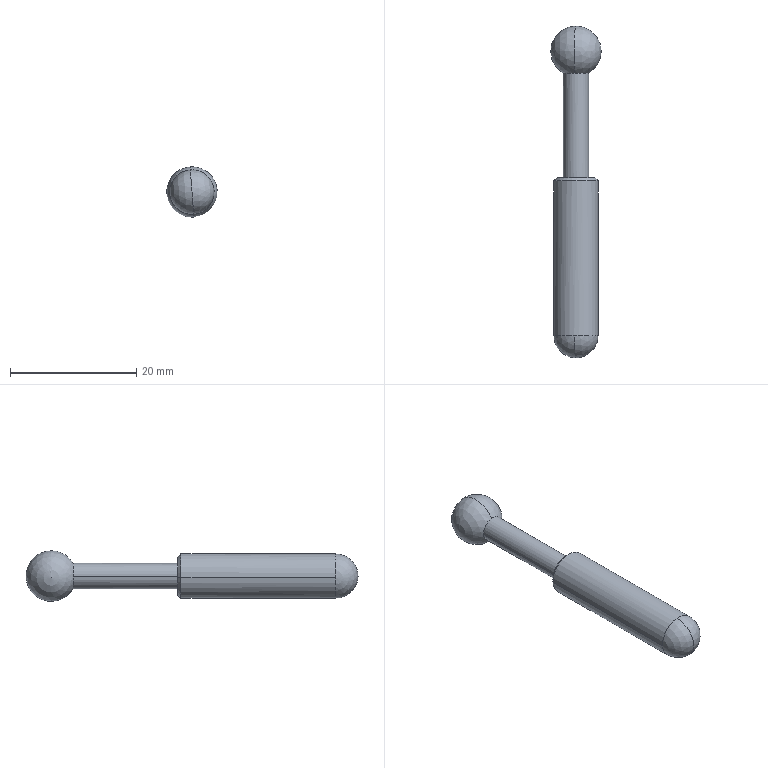Component | SolidWorks | GuidePost-1 | 1 solid | 11 faces | box 8 x 52.5 x 8 mm | volume 1522 mm3 | cylinder 4 | sphere 4 | cone 2 | plane 1 | commonest cylinder face diameters 4 x2 7 x2
build123d program:
from build123d import *

# Parameters (mm, degrees)
CHAMFER1_SIZE = 0.5


with BuildPart() as part:
    # Sketch1 → Revolve1 (revolve)
    with BuildSketch(Plane(origin=(0, 0, 0), x_dir=(0, 0, -1), z_dir=(1, 0, 0))):
        with BuildLine():
            Line((3.464, 2), (20, 2))
            Line((20, 2), (20, 3.5))
            Line((20, 3.5), (45, 3.5))
            ThreePointArc((45, 3.5), (47.475, 2.475), (48.5, 0))
            Line((48.5, 0), (-4, 0))
            ThreePointArc((-4, 0), (-1.035, 3.864), (3.464, 2))
        make_face()
    revolve(axis=Axis((0, 0, 4), (0, 0, -1)))

    # Chamfer1
    chamfer1_edges = [part.edges().sort_by_distance(p)[0] for p in [
        (0, -3.5, -20),
    ]]
    chamfer(chamfer1_edges, length=CHAMFER1_SIZE)


solid = part.part

# Placed as in the assembly
solid = solid.moved(Location((111.546, 64.028, 491.671), (-90, 0, 0)))
STEP:
#1=COLOUR_RGB('',0.7922,0.8196,0.9333);
#2=FILL_AREA_STYLE_COLOUR('',#1);
#3=FILL_AREA_STYLE('',(#2));
#4=SURFACE_STYLE_FILL_AREA(#3);
#5=SURFACE_SIDE_STYLE('',(#4));
#6=SURFACE_STYLE_USAGE(.BOTH.,#5);
#7=PRESENTATION_STYLE_ASSIGNMENT((#6));
#8=CARTESIAN_POINT('',(4.274,1.733,19.348));
#9=VERTEX_POINT('',#8);
#10=CARTESIAN_POINT('',(4.509,1.733,19.366));
#11=VERTEX_POINT('',#10);
#12=CARTESIAN_POINT('',(4.392,1.733,19.357));
#13=DIRECTION('',(0.,1.,0.));
#14=DIRECTION('',(0.9973,0.,0.07369));
#15=AXIS2_PLACEMENT_3D('',#12,#13,#14);
#16=CIRCLE('',#15,0.1181);
#17=EDGE_CURVE('',#9,#11,#16,.T.);
#18=ORIENTED_EDGE('',*,*,#17,.F.);
#19=CARTESIAN_POINT('',(4.254,1.714,19.347));
#20=VERTEX_POINT('',#19);
#21=CARTESIAN_POINT('',(4.274,1.733,19.348));
#22=DIRECTION('',(-0.7052,-0.7071,-0.05211));
#23=VECTOR('',#22,39.37);
#24=LINE('',#21,#23);
#25=EDGE_CURVE('',#9,#20,#24,.T.);
#26=ORIENTED_EDGE('',*,*,#25,.T.);
#27=CARTESIAN_POINT('',(4.529,1.714,19.367));
#28=VERTEX_POINT('',#27);
#29=CARTESIAN_POINT('',(4.392,1.714,19.357));
#30=DIRECTION('',(-0.,-1.,-0.));
#31=DIRECTION('',(0.9973,0.,0.07369));
#32=AXIS2_PLACEMENT_3D('',#29,#30,#31);
#33=CIRCLE('',#32,0.1378);
#34=EDGE_CURVE('',#28,#20,#33,.T.);
#35=ORIENTED_EDGE('',*,*,#34,.F.);
#36=CARTESIAN_POINT('',(4.509,1.733,19.366));
#37=DIRECTION('',(0.7052,-0.7071,0.05211));
#38=VECTOR('',#37,39.37);
#39=LINE('',#36,#38);
#40=EDGE_CURVE('',#11,#28,#39,.T.);
#41=ORIENTED_EDGE('',*,*,#40,.F.);
#42=EDGE_LOOP('',(#18,#26,#35,#41));
#43=FACE_OUTER_BOUND('',#42,.T.);
#44=CARTESIAN_POINT('',(4.392,1.733,19.357));
#45=DIRECTION('',(-0.,-1.,-0.));
#46=DIRECTION('',(0.9973,0.,0.07369));
#47=AXIS2_PLACEMENT_3D('',#44,#45,#46);
#48=CONICAL_SURFACE('',#47,0.1181,0.7854);
#49=ADVANCED_FACE('',(#43),#48,.T.);
#50=CARTESIAN_POINT('',(4.313,1.733,19.351));
#51=VERTEX_POINT('',#50);
#52=CARTESIAN_POINT('',(4.47,1.733,19.363));
#53=VERTEX_POINT('',#52);
#54=CARTESIAN_POINT('',(4.392,1.733,19.357));
#55=DIRECTION('',(0.,1.,0.));
#56=DIRECTION('',(-0.9973,0.,-0.07369));
#57=AXIS2_PLACEMENT_3D('',#54,#55,#56);
#58=CIRCLE('',#57,0.07874);
#59=EDGE_CURVE('',#51,#53,#58,.T.);
#60=ORIENTED_EDGE('',*,*,#59,.T.);
#61=CARTESIAN_POINT('',(4.47,2.384,19.363));
#62=VERTEX_POINT('',#61);
#63=CARTESIAN_POINT('',(4.47,2.678,19.363));
#64=DIRECTION('',(0.,1.,0.));
#65=VECTOR('',#64,39.37);
#66=LINE('',#63,#65);
#67=EDGE_CURVE('',#53,#62,#66,.T.);
#68=ORIENTED_EDGE('',*,*,#67,.T.);
#69=CARTESIAN_POINT('',(4.386,2.384,19.436));
#70=VERTEX_POINT('',#69);
#71=CARTESIAN_POINT('',(4.392,2.384,19.357));
#72=DIRECTION('',(0.,1.,0.));
#73=DIRECTION('',(-0.9973,0.,-0.07369));
#74=AXIS2_PLACEMENT_3D('',#71,#72,#73);
#75=CIRCLE('',#74,0.07874);
#76=EDGE_CURVE('',#70,#62,#75,.T.);
#77=ORIENTED_EDGE('',*,*,#76,.F.);
#78=CARTESIAN_POINT('',(4.313,2.384,19.351));
#79=VERTEX_POINT('',#78);
#80=CARTESIAN_POINT('',(4.392,2.384,19.357));
#81=DIRECTION('',(0.,1.,0.));
#82=DIRECTION('',(-0.9973,0.,-0.07369));
#83=AXIS2_PLACEMENT_3D('',#80,#81,#82);
#84=CIRCLE('',#83,0.07874);
#85=EDGE_CURVE('',#79,#70,#84,.T.);
#86=ORIENTED_EDGE('',*,*,#85,.F.);
#87=CARTESIAN_POINT('',(4.313,2.678,19.351));
#88=DIRECTION('',(0.,1.,0.));
#89=VECTOR('',#88,39.37);
#90=LINE('',#87,#89);
#91=EDGE_CURVE('',#51,#79,#90,.T.);
#92=ORIENTED_EDGE('',*,*,#91,.F.);
#93=EDGE_LOOP('',(#60,#68,#77,#86,#92));
#94=FACE_OUTER_BOUND('',#93,.T.);
#95=CARTESIAN_POINT('',(4.392,2.678,19.357));
#96=DIRECTION('',(0.,1.,0.));
#97=DIRECTION('',(-0.9973,0.,-0.07369));
#98=AXIS2_PLACEMENT_3D('',#95,#96,#97);
#99=CYLINDRICAL_SURFACE('',#98,0.07874);
#100=ADVANCED_FACE('',(#94),#99,.T.);
#101=CARTESIAN_POINT('',(4.381,0.7492,19.495));
#102=VERTEX_POINT('',#101);
#103=CARTESIAN_POINT('',(4.529,0.7492,19.367));
#104=VERTEX_POINT('',#103);
#105=CARTESIAN_POINT('',(4.392,0.7492,19.357));
#106=DIRECTION('',(0.,1.,0.));
#107=DIRECTION('',(-0.9973,0.,-0.07369));
#108=AXIS2_PLACEMENT_3D('',#105,#106,#107);
#109=CIRCLE('',#108,0.1378);
#110=EDGE_CURVE('',#102,#104,#109,.T.);
#111=ORIENTED_EDGE('',*,*,#110,.T.);
#112=CARTESIAN_POINT('',(4.529,2.678,19.367));
#113=DIRECTION('',(0.,1.,0.));
#114=VECTOR('',#113,39.37);
#115=LINE('',#112,#114);
#116=EDGE_CURVE('',#104,#28,#115,.T.);
#117=ORIENTED_EDGE('',*,*,#116,.T.);
#118=ORIENTED_EDGE('',*,*,#34,.T.);
#119=CARTESIAN_POINT('',(4.254,0.7492,19.347));
#120=VERTEX_POINT('',#119);
#121=CARTESIAN_POINT('',(4.254,2.678,19.347));
#122=DIRECTION('',(0.,1.,0.));
#123=VECTOR('',#122,39.37);
#124=LINE('',#121,#123);
#125=EDGE_CURVE('',#120,#20,#124,.T.);
#126=ORIENTED_EDGE('',*,*,#125,.F.);
#127=CARTESIAN_POINT('',(4.392,0.7492,19.357));
#128=DIRECTION('',(0.,1.,0.));
#129=DIRECTION('',(-0.9973,0.,-0.07369));
#130=AXIS2_PLACEMENT_3D('',#127,#128,#129);
#131=CIRCLE('',#130,0.1378);
#132=EDGE_CURVE('',#120,#102,#131,.T.);
#133=ORIENTED_EDGE('',*,*,#132,.T.);
#134=EDGE_LOOP('',(#111,#117,#118,#126,#133));
#135=FACE_OUTER_BOUND('',#134,.T.);
#136=CARTESIAN_POINT('',(4.392,2.678,19.357));
#137=DIRECTION('',(0.,1.,0.));
#138=DIRECTION('',(-0.9973,0.,-0.07369));
#139=AXIS2_PLACEMENT_3D('',#136,#137,#138);
#140=CYLINDRICAL_SURFACE('',#139,0.1378);
#141=ADVANCED_FACE('',(#135),#140,.T.);
#142=CARTESIAN_POINT('',(4.392,0.6114,19.357));
#143=VERTEX_POINT('',#142);
#144=CARTESIAN_POINT('',(4.392,0.7492,19.357));
#145=DIRECTION('',(-0.9973,0.,-0.07369));
#146=DIRECTION('',(-0.07369,0.,0.9973));
#147=AXIS2_PLACEMENT_3D('',#144,#145,#146);
#148=CIRCLE('',#147,0.1378);
#149=EDGE_CURVE('',#143,#102,#148,.T.);
#150=ORIENTED_EDGE('',*,*,#149,.F.);
#151=CARTESIAN_POINT('',(4.402,0.7492,19.22));
#152=VERTEX_POINT('',#151);
#153=CARTESIAN_POINT('',(4.392,0.7492,19.357));
#154=DIRECTION('',(0.9973,-0.,0.07369));
#155=DIRECTION('',(0.07369,0.,-0.9973));
#156=AXIS2_PLACEMENT_3D('',#153,#154,#155);
#157=CIRCLE('',#156,0.1378);
#158=EDGE_CURVE('',#143,#152,#157,.T.);
#159=ORIENTED_EDGE('',*,*,#158,.T.);
#160=CARTESIAN_POINT('',(4.392,0.7492,19.357));
#161=DIRECTION('',(0.,1.,0.));
#162=DIRECTION('',(-0.9973,0.,-0.07369));
#163=AXIS2_PLACEMENT_3D('',#160,#161,#162);
#164=CIRCLE('',#163,0.1378);
#165=EDGE_CURVE('',#104,#152,#164,.T.);
#166=ORIENTED_EDGE('',*,*,#165,.F.);
#167=ORIENTED_EDGE('',*,*,#110,.F.);
#168=EDGE_LOOP('',(#150,#159,#166,#167));
#169=FACE_OUTER_BOUND('',#168,.T.);
#170=CARTESIAN_POINT('',(4.392,0.7492,19.357));
#171=DIRECTION('',(0.9973,-0.,0.07369));
#172=DIRECTION('',(-0.07369,0.,0.9973));
#173=AXIS2_PLACEMENT_3D('',#170,#171,#172);
#174=SPHERICAL_SURFACE('',#173,0.1378);
#175=ADVANCED_FACE('',(#169),#174,.T.);
#176=ORIENTED_EDGE('',*,*,#76,.T.);
#177=CARTESIAN_POINT('',(4.397,2.384,19.279));
#178=VERTEX_POINT('',#177);
#179=CARTESIAN_POINT('',(4.392,2.384,19.357));
#180=DIRECTION('',(0.,1.,0.));
#181=DIRECTION('',(-0.9973,0.,-0.07369));
#182=AXIS2_PLACEMENT_3D('',#179,#180,#181);
#183=CIRCLE('',#182,0.07874);
#184=EDGE_CURVE('',#62,#178,#183,.T.);
#185=ORIENTED_EDGE('',*,*,#184,.T.);
#186=CARTESIAN_POINT('',(4.392,2.678,19.357));
#187=VERTEX_POINT('',#186);
#188=CARTESIAN_POINT('',(4.392,2.521,19.357));
#189=DIRECTION('',(0.9973,-0.,0.07369));
#190=DIRECTION('',(0.07369,0.,-0.9973));
#191=AXIS2_PLACEMENT_3D('',#188,#189,#190);
#192=CIRCLE('',#191,0.1575);
#193=EDGE_CURVE('',#178,#187,#192,.T.);
#194=ORIENTED_EDGE('',*,*,#193,.T.);
#195=CARTESIAN_POINT('',(4.392,2.521,19.357));
#196=DIRECTION('',(-0.9973,0.,-0.07369));
#197=DIRECTION('',(-0.07369,0.,0.9973));
#198=AXIS2_PLACEMENT_3D('',#195,#196,#197);
#199=CIRCLE('',#198,0.1575);
#200=EDGE_CURVE('',#70,#187,#199,.T.);
#201=ORIENTED_EDGE('',*,*,#200,.F.);
#202=EDGE_LOOP('',(#176,#185,#194,#201));
#203=FACE_OUTER_BOUND('',#202,.T.);
#204=CARTESIAN_POINT('',(4.392,2.521,19.357));
#205=DIRECTION('',(0.9973,-0.,0.07369));
#206=DIRECTION('',(-0.07369,0.,0.9973));
#207=AXIS2_PLACEMENT_3D('',#204,#205,#206);
#208=SPHERICAL_SURFACE('',#207,0.1575);
#209=ADVANCED_FACE('',(#203),#208,.T.);
#210=ORIENTED_EDGE('',*,*,#193,.F.);
#211=CARTESIAN_POINT('',(4.392,2.384,19.357));
#212=DIRECTION('',(0.,1.,0.));
#213=DIRECTION('',(-0.9973,0.,-0.07369));
#214=AXIS2_PLACEMENT_3D('',#211,#212,#213);
#215=CIRCLE('',#214,0.07874);
#216=EDGE_CURVE('',#178,#79,#215,.T.);
#217=ORIENTED_EDGE('',*,*,#216,.T.);
#218=ORIENTED_EDGE('',*,*,#85,.T.);
#219=ORIENTED_EDGE('',*,*,#200,.T.);
#220=EDGE_LOOP('',(#210,#217,#218,#219));
#221=FACE_OUTER_BOUND('',#220,.T.);
#222=CARTESIAN_POINT('',(4.392,2.521,19.357));
#223=DIRECTION('',(0.9973,-0.,0.07369));
#224=DIRECTION('',(-0.07369,0.,0.9973));
#225=AXIS2_PLACEMENT_3D('',#222,#223,#224);
#226=SPHERICAL_SURFACE('',#225,0.1575);
#227=ADVANCED_FACE('',(#221),#226,.T.);
#228=ORIENTED_EDGE('',*,*,#158,.F.);
#229=ORIENTED_EDGE('',*,*,#149,.T.);
#230=ORIENTED_EDGE('',*,*,#132,.F.);
#231=CARTESIAN_POINT('',(4.392,0.7492,19.357));
#232=DIRECTION('',(0.,1.,0.));
#233=DIRECTION('',(-0.9973,0.,-0.07369));
#234=AXIS2_PLACEMENT_3D('',#231,#232,#233);
#235=CIRCLE('',#234,0.1378);
#236=EDGE_CURVE('',#152,#120,#235,.T.);
#237=ORIENTED_EDGE('',*,*,#236,.F.);
#238=EDGE_LOOP('',(#228,#229,#230,#237));
#239=FACE_OUTER_BOUND('',#238,.T.);
#240=CARTESIAN_POINT('',(4.392,0.7492,19.357));
#241=DIRECTION('',(0.9973,-0.,0.07369));
#242=DIRECTION('',(-0.07369,0.,0.9973));
#243=AXIS2_PLACEMENT_3D('',#240,#241,#242);
#244=SPHERICAL_SURFACE('',#243,0.1378);
#245=ADVANCED_FACE('',(#239),#244,.T.);
#246=ORIENTED_EDGE('',*,*,#116,.F.);
#247=ORIENTED_EDGE('',*,*,#165,.T.);
#248=ORIENTED_EDGE('',*,*,#236,.T.);
#249=ORIENTED_EDGE('',*,*,#125,.T.);
#250=CARTESIAN_POINT('',(4.392,1.714,19.357));
#251=DIRECTION('',(-0.,-1.,-0.));
#252=DIRECTION('',(0.9973,0.,0.07369));
#253=AXIS2_PLACEMENT_3D('',#250,#251,#252);
#254=CIRCLE('',#253,0.1378);
#255=EDGE_CURVE('',#20,#28,#254,.T.);
#256=ORIENTED_EDGE('',*,*,#255,.T.);
#257=EDGE_LOOP('',(#246,#247,#248,#249,#256));
#258=FACE_OUTER_BOUND('',#257,.T.);
#259=CARTESIAN_POINT('',(4.392,2.678,19.357));
#260=DIRECTION('',(0.,1.,0.));
#261=DIRECTION('',(-0.9973,0.,-0.07369));
#262=AXIS2_PLACEMENT_3D('',#259,#260,#261);
#263=CYLINDRICAL_SURFACE('',#262,0.1378);
#264=ADVANCED_FACE('',(#258),#263,.T.);
#265=CARTESIAN_POINT('',(4.392,1.733,19.357));
#266=DIRECTION('',(0.,1.,0.));
#267=DIRECTION('',(0.9973,0.,0.07369));
#268=AXIS2_PLACEMENT_3D('',#265,#266,#267);
#269=CIRCLE('',#268,0.1181);
#270=EDGE_CURVE('',#11,#9,#269,.T.);
#271=ORIENTED_EDGE('',*,*,#270,.T.);
#272=ORIENTED_EDGE('',*,*,#17,.T.);
#273=EDGE_LOOP('',(#271,#272));
#274=FACE_OUTER_BOUND('',#273,.T.);
#275=ORIENTED_EDGE('',*,*,#59,.F.);
#276=CARTESIAN_POINT('',(4.392,1.733,19.357));
#277=DIRECTION('',(0.,1.,0.));
#278=DIRECTION('',(-0.9973,0.,-0.07369));
#279=AXIS2_PLACEMENT_3D('',#276,#277,#278);
#280=CIRCLE('',#279,0.07874);
#281=EDGE_CURVE('',#53,#51,#280,.T.);
#282=ORIENTED_EDGE('',*,*,#281,.F.);
#283=EDGE_LOOP('',(#275,#282));
#284=FACE_BOUND('',#283,.T.);
#285=CARTESIAN_POINT('',(4.386,1.733,19.436));
#286=DIRECTION('',(-0.,-1.,-0.));
#287=DIRECTION('',(0.9973,-0.,0.07369));
#288=AXIS2_PLACEMENT_3D('',#285,#286,#287);
#289=PLANE('',#288);
#290=ADVANCED_FACE('',(#274,#284),#289,.F.);
#291=ORIENTED_EDGE('',*,*,#67,.F.);
#292=ORIENTED_EDGE('',*,*,#281,.T.);
#293=ORIENTED_EDGE('',*,*,#91,.T.);
#294=ORIENTED_EDGE('',*,*,#216,.F.);
#295=ORIENTED_EDGE('',*,*,#184,.F.);
#296=EDGE_LOOP('',(#291,#292,#293,#294,#295));
#297=FACE_OUTER_BOUND('',#296,.T.);
#298=CARTESIAN_POINT('',(4.392,2.678,19.357));
#299=DIRECTION('',(0.,1.,0.));
#300=DIRECTION('',(-0.9973,0.,-0.07369));
#301=AXIS2_PLACEMENT_3D('',#298,#299,#300);
#302=CYLINDRICAL_SURFACE('',#301,0.07874);
#303=ADVANCED_FACE('',(#297),#302,.T.);
#304=ORIENTED_EDGE('',*,*,#25,.F.);
#305=ORIENTED_EDGE('',*,*,#270,.F.);
#306=ORIENTED_EDGE('',*,*,#40,.T.);
#307=ORIENTED_EDGE('',*,*,#255,.F.);
#308=EDGE_LOOP('',(#304,#305,#306,#307));
#309=FACE_OUTER_BOUND('',#308,.T.);
#310=CARTESIAN_POINT('',(4.392,1.733,19.357));
#311=DIRECTION('',(-0.,-1.,-0.));
#312=DIRECTION('',(0.9973,0.,0.07369));
#313=AXIS2_PLACEMENT_3D('',#310,#311,#312);
#314=CONICAL_SURFACE('',#313,0.1181,0.7854);
#315=ADVANCED_FACE('',(#309),#314,.T.);
#316=CLOSED_SHELL('',(#49,#100,#141,#175,#209,#227,#245,#264,#290,#303,#315));
#317=MANIFOLD_SOLID_BREP('',#316);
#318=STYLED_ITEM('',(#7),#317);
#319=PRESENTATION_LAYER_ASSIGNMENT('','',(#318));
#320=CARTESIAN_POINT('',(0.,0.,0.));
#321=DIRECTION('',(0.,0.,1.));
#322=DIRECTION('',(1.,0.,0.));
#323=AXIS2_PLACEMENT_3D('',#320,#321,#322);
#324=(LENGTH_UNIT()NAMED_UNIT(*)SI_UNIT($,.METRE.));
#325=LENGTH_MEASURE_WITH_UNIT(LENGTH_MEASURE(0.0254),#324);
#326=DIMENSIONAL_EXPONENTS(1.,0.,0.,0.,0.,0.,0.);
#327=(CONVERSION_BASED_UNIT('',#325)LENGTH_UNIT()NAMED_UNIT(#326));
#328=UNCERTAINTY_MEASURE_WITH_UNIT(LENGTH_MEASURE(0.00001),#327,'','');
#329=(NAMED_UNIT(*)PLANE_ANGLE_UNIT()SI_UNIT($,.RADIAN.));
#330=(NAMED_UNIT(*)SI_UNIT($,.STERADIAN.)SOLID_ANGLE_UNIT());
#331=(GEOMETRIC_REPRESENTATION_CONTEXT(3)GLOBAL_UNCERTAINTY_ASSIGNED_CONTEXT((#328))GLOBAL_UNIT_ASSIGNED_CONTEXT((#327,#329,#330))REPRESENTATION_CONTEXT('',''));
#332=ADVANCED_BREP_SHAPE_REPRESENTATION('',(#317,#323),#331);
#333=(LENGTH_UNIT()NAMED_UNIT(*)SI_UNIT($,.METRE.));
#334=LENGTH_MEASURE_WITH_UNIT(LENGTH_MEASURE(0.0254),#333);
#335=DIMENSIONAL_EXPONENTS(1.,0.,0.,0.,0.,0.,0.);
#336=(CONVERSION_BASED_UNIT('',#334)LENGTH_UNIT()NAMED_UNIT(#335));
#337=UNCERTAINTY_MEASURE_WITH_UNIT(LENGTH_MEASURE(0.00001),#336,'','');
#338=(NAMED_UNIT(*)PLANE_ANGLE_UNIT()SI_UNIT($,.RADIAN.));
#339=(NAMED_UNIT(*)SI_UNIT($,.STERADIAN.)SOLID_ANGLE_UNIT());
#340=(GEOMETRIC_REPRESENTATION_CONTEXT(3)GLOBAL_UNCERTAINTY_ASSIGNED_CONTEXT((#337))GLOBAL_UNIT_ASSIGNED_CONTEXT((#336,#338,#339))REPRESENTATION_CONTEXT('',''));
#341=MECHANICAL_DESIGN_GEOMETRIC_PRESENTATION_REPRESENTATION('',(#318),#340);